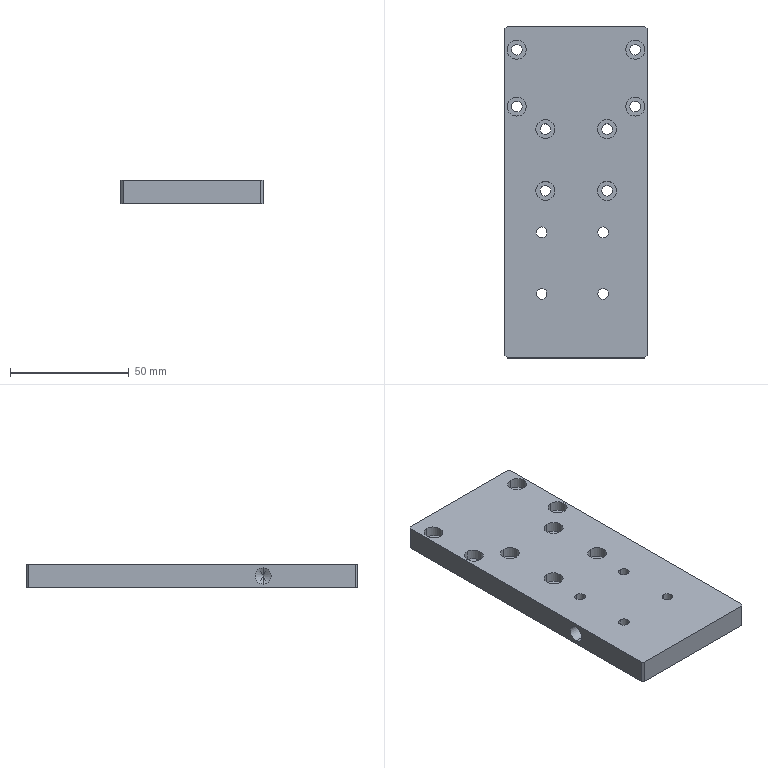Component | SolidWorks | CCDJSLiftingCylinderFixingPlate01-1 | 1 solid | 90 faces | box 60 x 140 x 10 mm | volume 78215 mm3 | cylinder 58 | plane 22 | cone 10 | commonest cylinder face diameters 8 x26 4.5 x24 3.3 x6 6.8 x2
build123d program:
from build123d import *

# Parameters (mm, degrees)
SKETCH1_W                                       = 140
SKETCH1_H                                       = 60
BOSS_EXTRUDE1_DEPTH                             = 10
M8_TAPPED_HOLE1_D                               = 6.8
M8_TAPPED_HOLE1_DEPTH                           = 19.75
M8_TAPPED_HOLE1_TIP                             = 2.043
M4_TAPPED_HOLE1_D                               = 3.3
M4_TAPPED_HOLE1_DEPTH                           = 10.1
M4_TAPPED_HOLE1_TIP                             = 0.9914
M4_HEX_SOCKET_HEAD_CAP_SCREW_CBORE1_D           = 4.5
M4_HEX_SOCKET_HEAD_CAP_SCREW_CBORE1_DEPTH       = 10.1
M4_HEX_SOCKET_HEAD_CAP_SCREW_CBORE1_CBORE_D     = 8
M4_HEX_SOCKET_HEAD_CAP_SCREW_CBORE1_CBORE_DEPTH = 4.4
M4_HEX_SOCKET_HEAD_CAP_SCREW_CBORE1_TIP         = 1.352
M4_HEX_SOCKET_HEAD_CAP_SCREW_CBORE2_D           = 4.5
M4_HEX_SOCKET_HEAD_CAP_SCREW_CBORE2_DEPTH       = 10.1
M4_HEX_SOCKET_HEAD_CAP_SCREW_CBORE2_CBORE_D     = 8
M4_HEX_SOCKET_HEAD_CAP_SCREW_CBORE2_CBORE_DEPTH = 4.4
M4_HEX_SOCKET_HEAD_CAP_SCREW_CBORE2_TIP         = 1.352
M4_HEX_SOCKET_HEAD_CAP_SCREW_CBORE3_D           = 4.5
M4_HEX_SOCKET_HEAD_CAP_SCREW_CBORE3_DEPTH       = 10.1
M4_HEX_SOCKET_HEAD_CAP_SCREW_CBORE3_CBORE_D     = 8
M4_HEX_SOCKET_HEAD_CAP_SCREW_CBORE3_CBORE_DEPTH = 4.4
M4_HEX_SOCKET_HEAD_CAP_SCREW_CBORE3_TIP         = 1.352
M8_TAPPED_HOLE2_D                               = 8
M8_TAPPED_HOLE2_DEPTH                           = 19.75
M8_TAPPED_HOLE2_TIP                             = 2.403
CHAMFER1_SIZE                                   = 1


with BuildPart() as part:
    # Sketch1 → Boss-Extrude1 (new body)
    with BuildSketch(Plane.XY):
        Rectangle(SKETCH1_W, SKETCH1_H)
    extrude(amount=BOSS_EXTRUDE1_DEPTH)

    # M8 Tapped Hole1
    with Locations(Plane(origin=(0, -30, 0), x_dir=(-1, 0, 0), z_dir=(0, -1, 0))):
        with Locations((-30, -5)):
            Hole(M8_TAPPED_HOLE1_D / 2, depth=M8_TAPPED_HOLE1_DEPTH)
            with Locations((0, 0, -(M8_TAPPED_HOLE1_DEPTH + M8_TAPPED_HOLE1_TIP / 2))):  # 118° drill point
                Cone(0, M8_TAPPED_HOLE1_D / 2, M8_TAPPED_HOLE1_TIP, mode=Mode.SUBTRACT)

    # M4 Tapped Hole1
    with Locations(Plane.ZY.offset(70)):
        with Locations((5, 15), (5, 0), (5, -15)):
            Hole(M4_TAPPED_HOLE1_D / 2, depth=M4_TAPPED_HOLE1_DEPTH)
            with Locations((0, 0, -(M4_TAPPED_HOLE1_DEPTH + M4_TAPPED_HOLE1_TIP / 2))):  # 118° drill point
                Cone(0, M4_TAPPED_HOLE1_D / 2, M4_TAPPED_HOLE1_TIP, mode=Mode.SUBTRACT)

    # M4 Hex Socket Head Cap Screw CBORE1
    with Locations(Plane.XY.offset(10)):
        with Locations((-60, -25), (-36, -25), (-60, 25), (-36, 25)):
            CounterBoreHole(M4_HEX_SOCKET_HEAD_CAP_SCREW_CBORE1_D / 2, M4_HEX_SOCKET_HEAD_CAP_SCREW_CBORE1_CBORE_D / 2, M4_HEX_SOCKET_HEAD_CAP_SCREW_CBORE1_CBORE_DEPTH, depth=M4_HEX_SOCKET_HEAD_CAP_SCREW_CBORE1_DEPTH)
            with Locations((0, 0, -(M4_HEX_SOCKET_HEAD_CAP_SCREW_CBORE1_DEPTH + M4_HEX_SOCKET_HEAD_CAP_SCREW_CBORE1_TIP / 2))):  # 118° drill point
                Cone(0, M4_HEX_SOCKET_HEAD_CAP_SCREW_CBORE1_D / 2, M4_HEX_SOCKET_HEAD_CAP_SCREW_CBORE1_TIP, mode=Mode.SUBTRACT)

    # M4 Hex Socket Head Cap Screw CBORE2
    with Locations(Plane.XY.offset(10)):
        with Locations((-26.5, -12.9), (-26.5, 13.1), (-0.5, 13.1), (-0.5, -12.9)):
            CounterBoreHole(M4_HEX_SOCKET_HEAD_CAP_SCREW_CBORE2_D / 2, M4_HEX_SOCKET_HEAD_CAP_SCREW_CBORE2_CBORE_D / 2, M4_HEX_SOCKET_HEAD_CAP_SCREW_CBORE2_CBORE_DEPTH, depth=M4_HEX_SOCKET_HEAD_CAP_SCREW_CBORE2_DEPTH)
            with Locations((0, 0, -(M4_HEX_SOCKET_HEAD_CAP_SCREW_CBORE2_DEPTH + M4_HEX_SOCKET_HEAD_CAP_SCREW_CBORE2_TIP / 2))):  # 118° drill point
                Cone(0, M4_HEX_SOCKET_HEAD_CAP_SCREW_CBORE2_D / 2, M4_HEX_SOCKET_HEAD_CAP_SCREW_CBORE2_TIP, mode=Mode.SUBTRACT)

    # M4 Hex Socket Head Cap Screw CBORE3
    with Locations(Plane(origin=(0, 0, 0), x_dir=(-1, 0, 0), z_dir=(0, 0, -1))):
        with Locations((-17, 11.5), (-43, 11.5), (-17, -14.5), (-43, -14.5)):
            CounterBoreHole(M4_HEX_SOCKET_HEAD_CAP_SCREW_CBORE3_D / 2, M4_HEX_SOCKET_HEAD_CAP_SCREW_CBORE3_CBORE_D / 2, M4_HEX_SOCKET_HEAD_CAP_SCREW_CBORE3_CBORE_DEPTH, depth=M4_HEX_SOCKET_HEAD_CAP_SCREW_CBORE3_DEPTH)
            with Locations((0, 0, -(M4_HEX_SOCKET_HEAD_CAP_SCREW_CBORE3_DEPTH + M4_HEX_SOCKET_HEAD_CAP_SCREW_CBORE3_TIP / 2))):  # 118° drill point
                Cone(0, M4_HEX_SOCKET_HEAD_CAP_SCREW_CBORE3_D / 2, M4_HEX_SOCKET_HEAD_CAP_SCREW_CBORE3_TIP, mode=Mode.SUBTRACT)

    # M8 Tapped Hole2
    with Locations(Plane(origin=(0, 30, 0), x_dir=(1, 0, 0), z_dir=(0, 1, 0))):
        with Locations((30, -5)):
            Hole(M8_TAPPED_HOLE2_D / 2, depth=M8_TAPPED_HOLE2_DEPTH)
            with Locations((0, 0, -(M8_TAPPED_HOLE2_DEPTH + M8_TAPPED_HOLE2_TIP / 2))):  # 118° drill point
                Cone(0, M8_TAPPED_HOLE2_D / 2, M8_TAPPED_HOLE2_TIP, mode=Mode.SUBTRACT)

    # Chamfer1
    chamfer1_edges = [part.edges().sort_by_distance(p)[0] for p in [
        (70, -30, 5),
        (-70, -30, 5),
        (-70, 30, 5),
        (70, 30, 5),
    ]]
    chamfer(chamfer1_edges, length=CHAMFER1_SIZE)


solid = part.part

# Placed as in the assembly
solid = solid.moved(Location((-159, 456.564, -68.57), (0, 0, -90)))